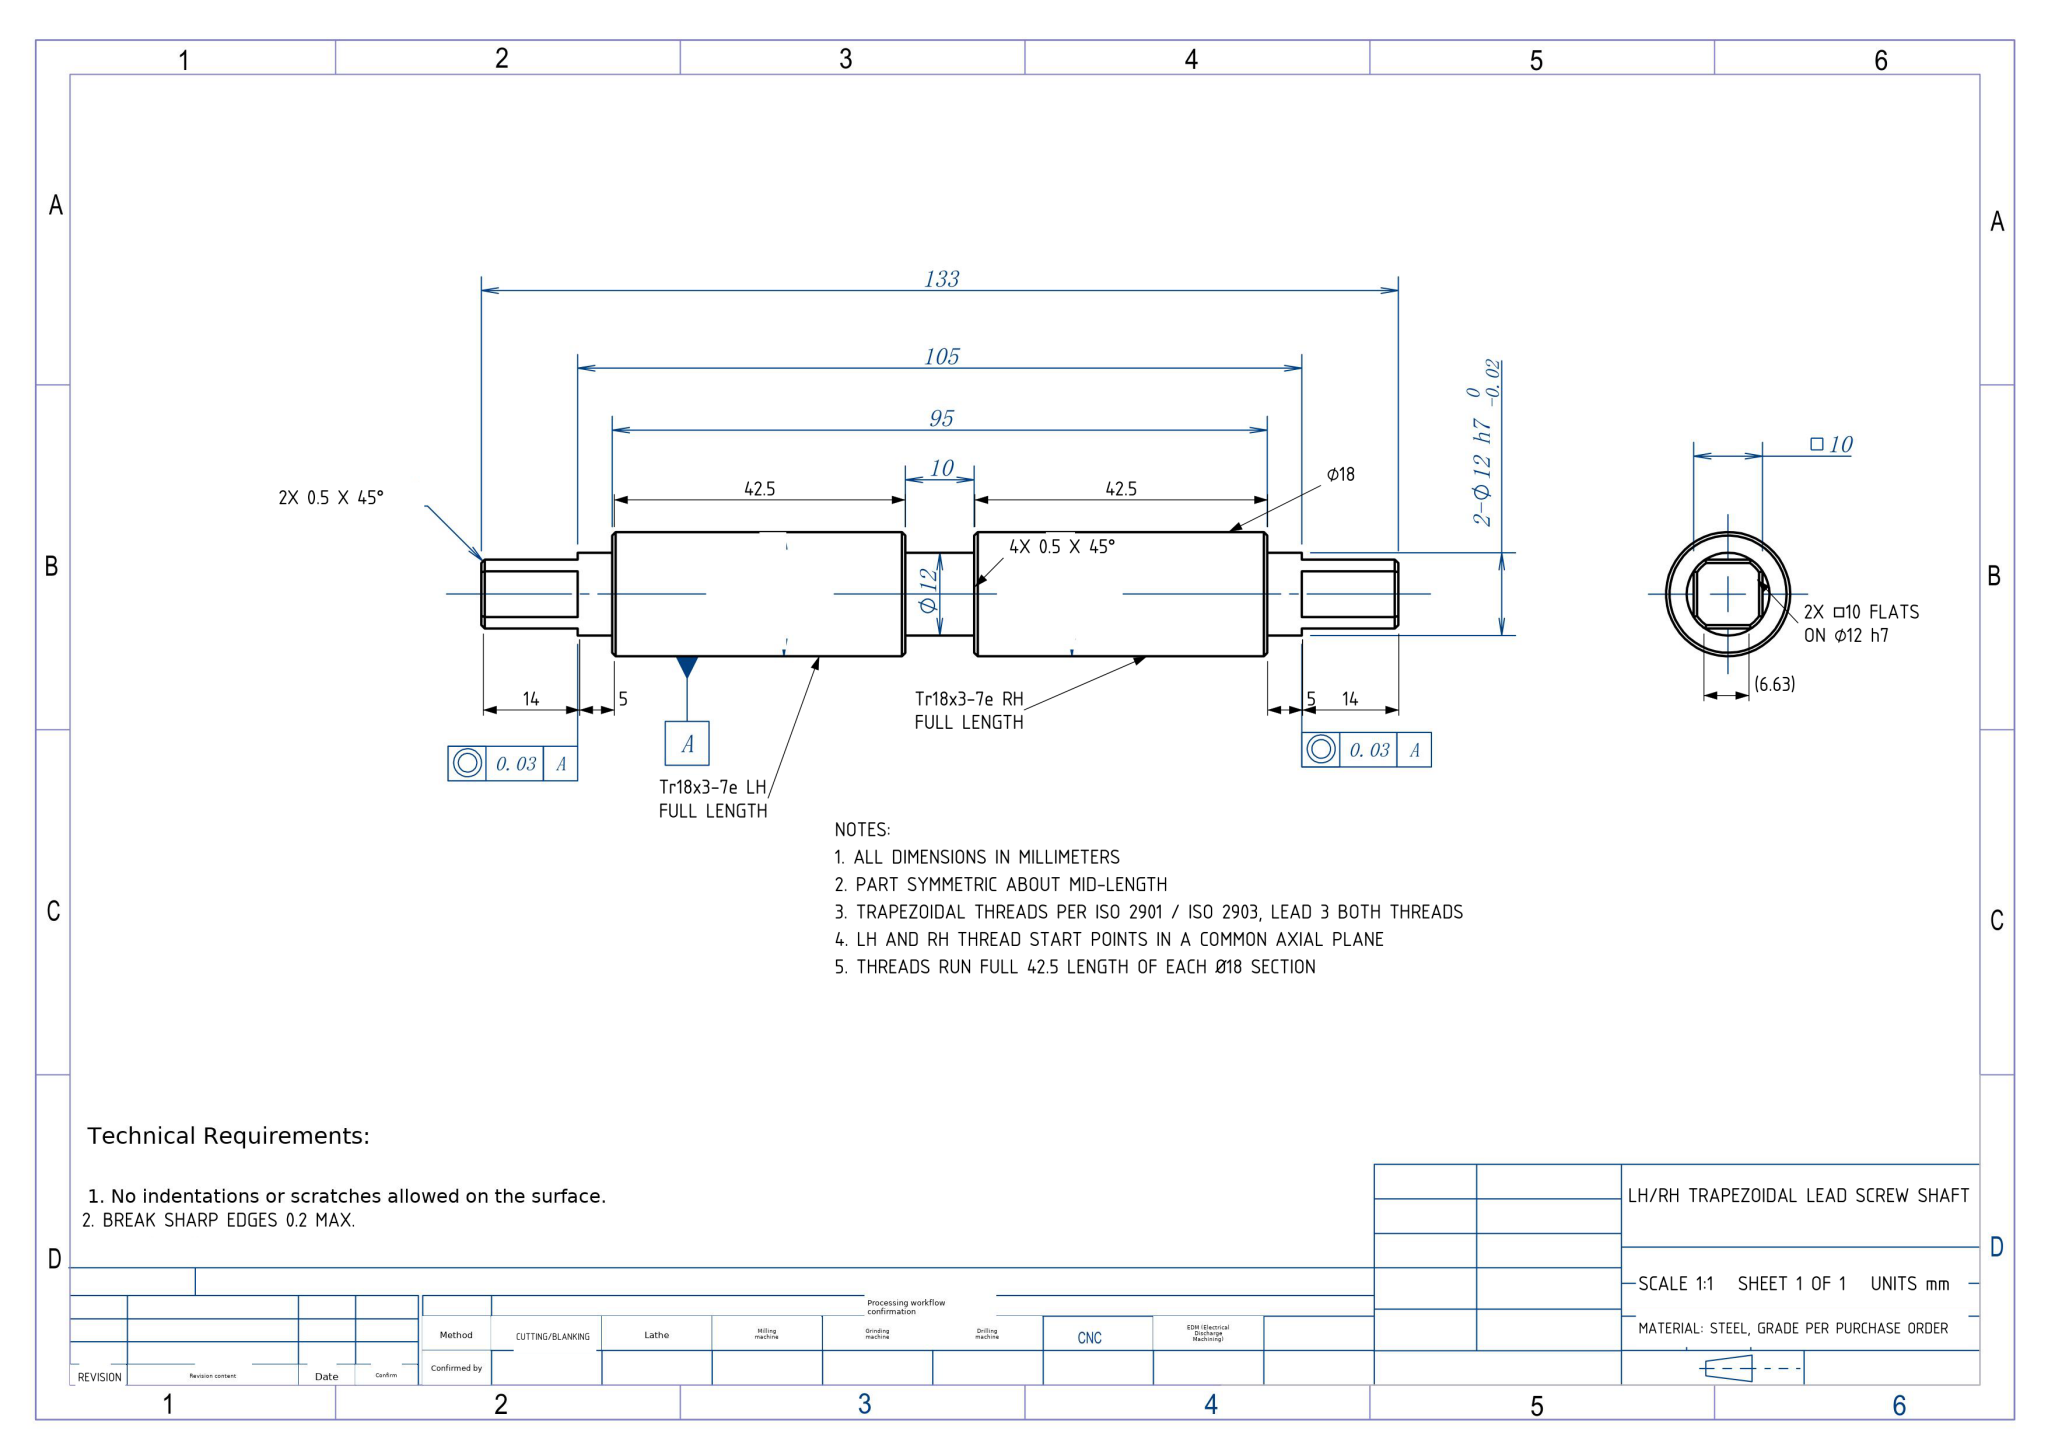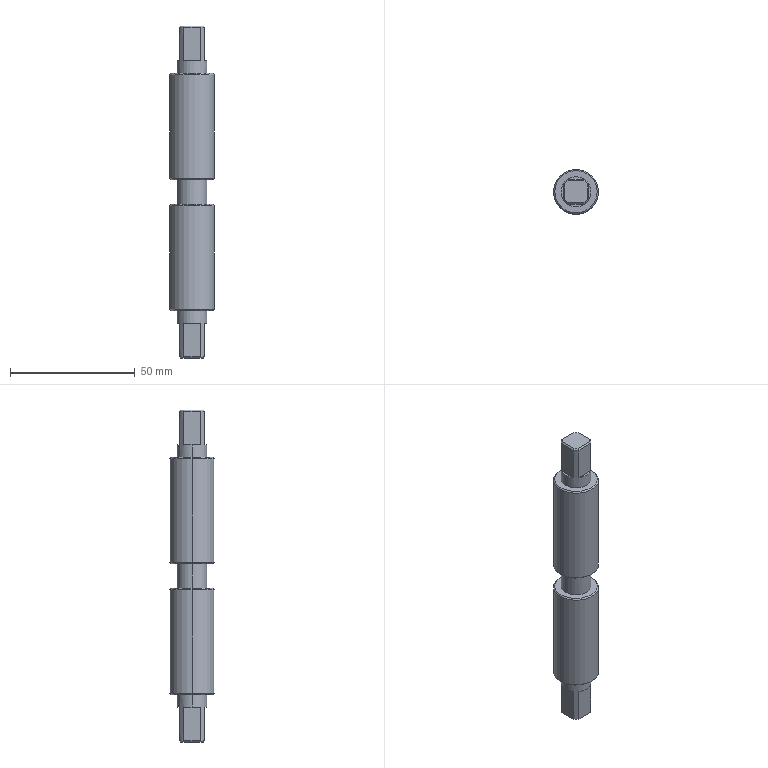Part | NX | mm | 1 solid | 56 faces | box 18 x 18 x 133 mm | volume 26518 mm3 | plane 30 | cone 16 | cylinder 10 | commonest cylinder face diameters 12 x6 18 x4